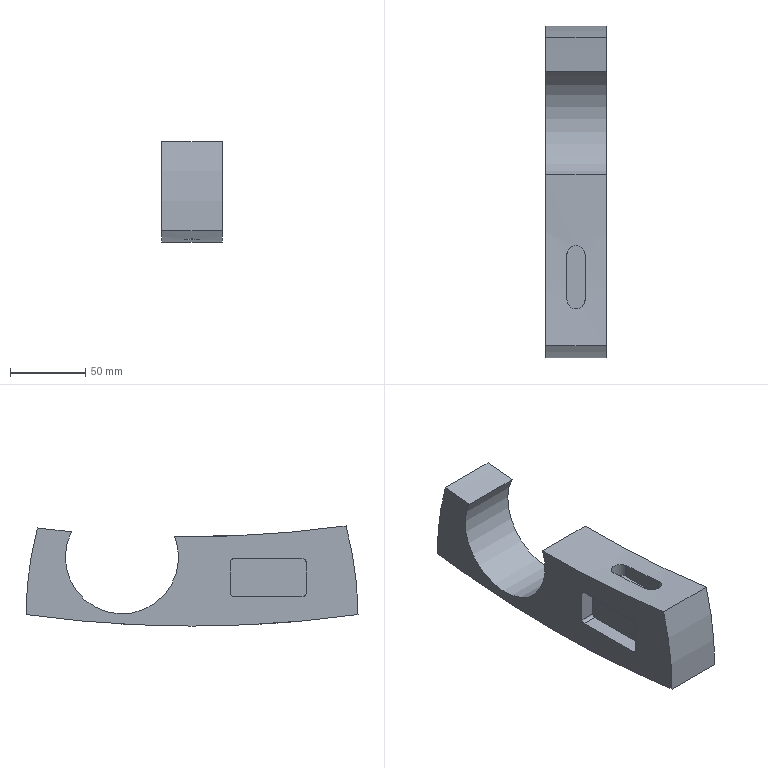Component | NX | BODY1 | 1 solid | 32 faces | volume 358482 mm3 | cylinder 17 | plane 15 | commonest cylinder face diameters 4 x4 1600 x3 8 x3 460 x2 12 x2 10 x2 75 x1